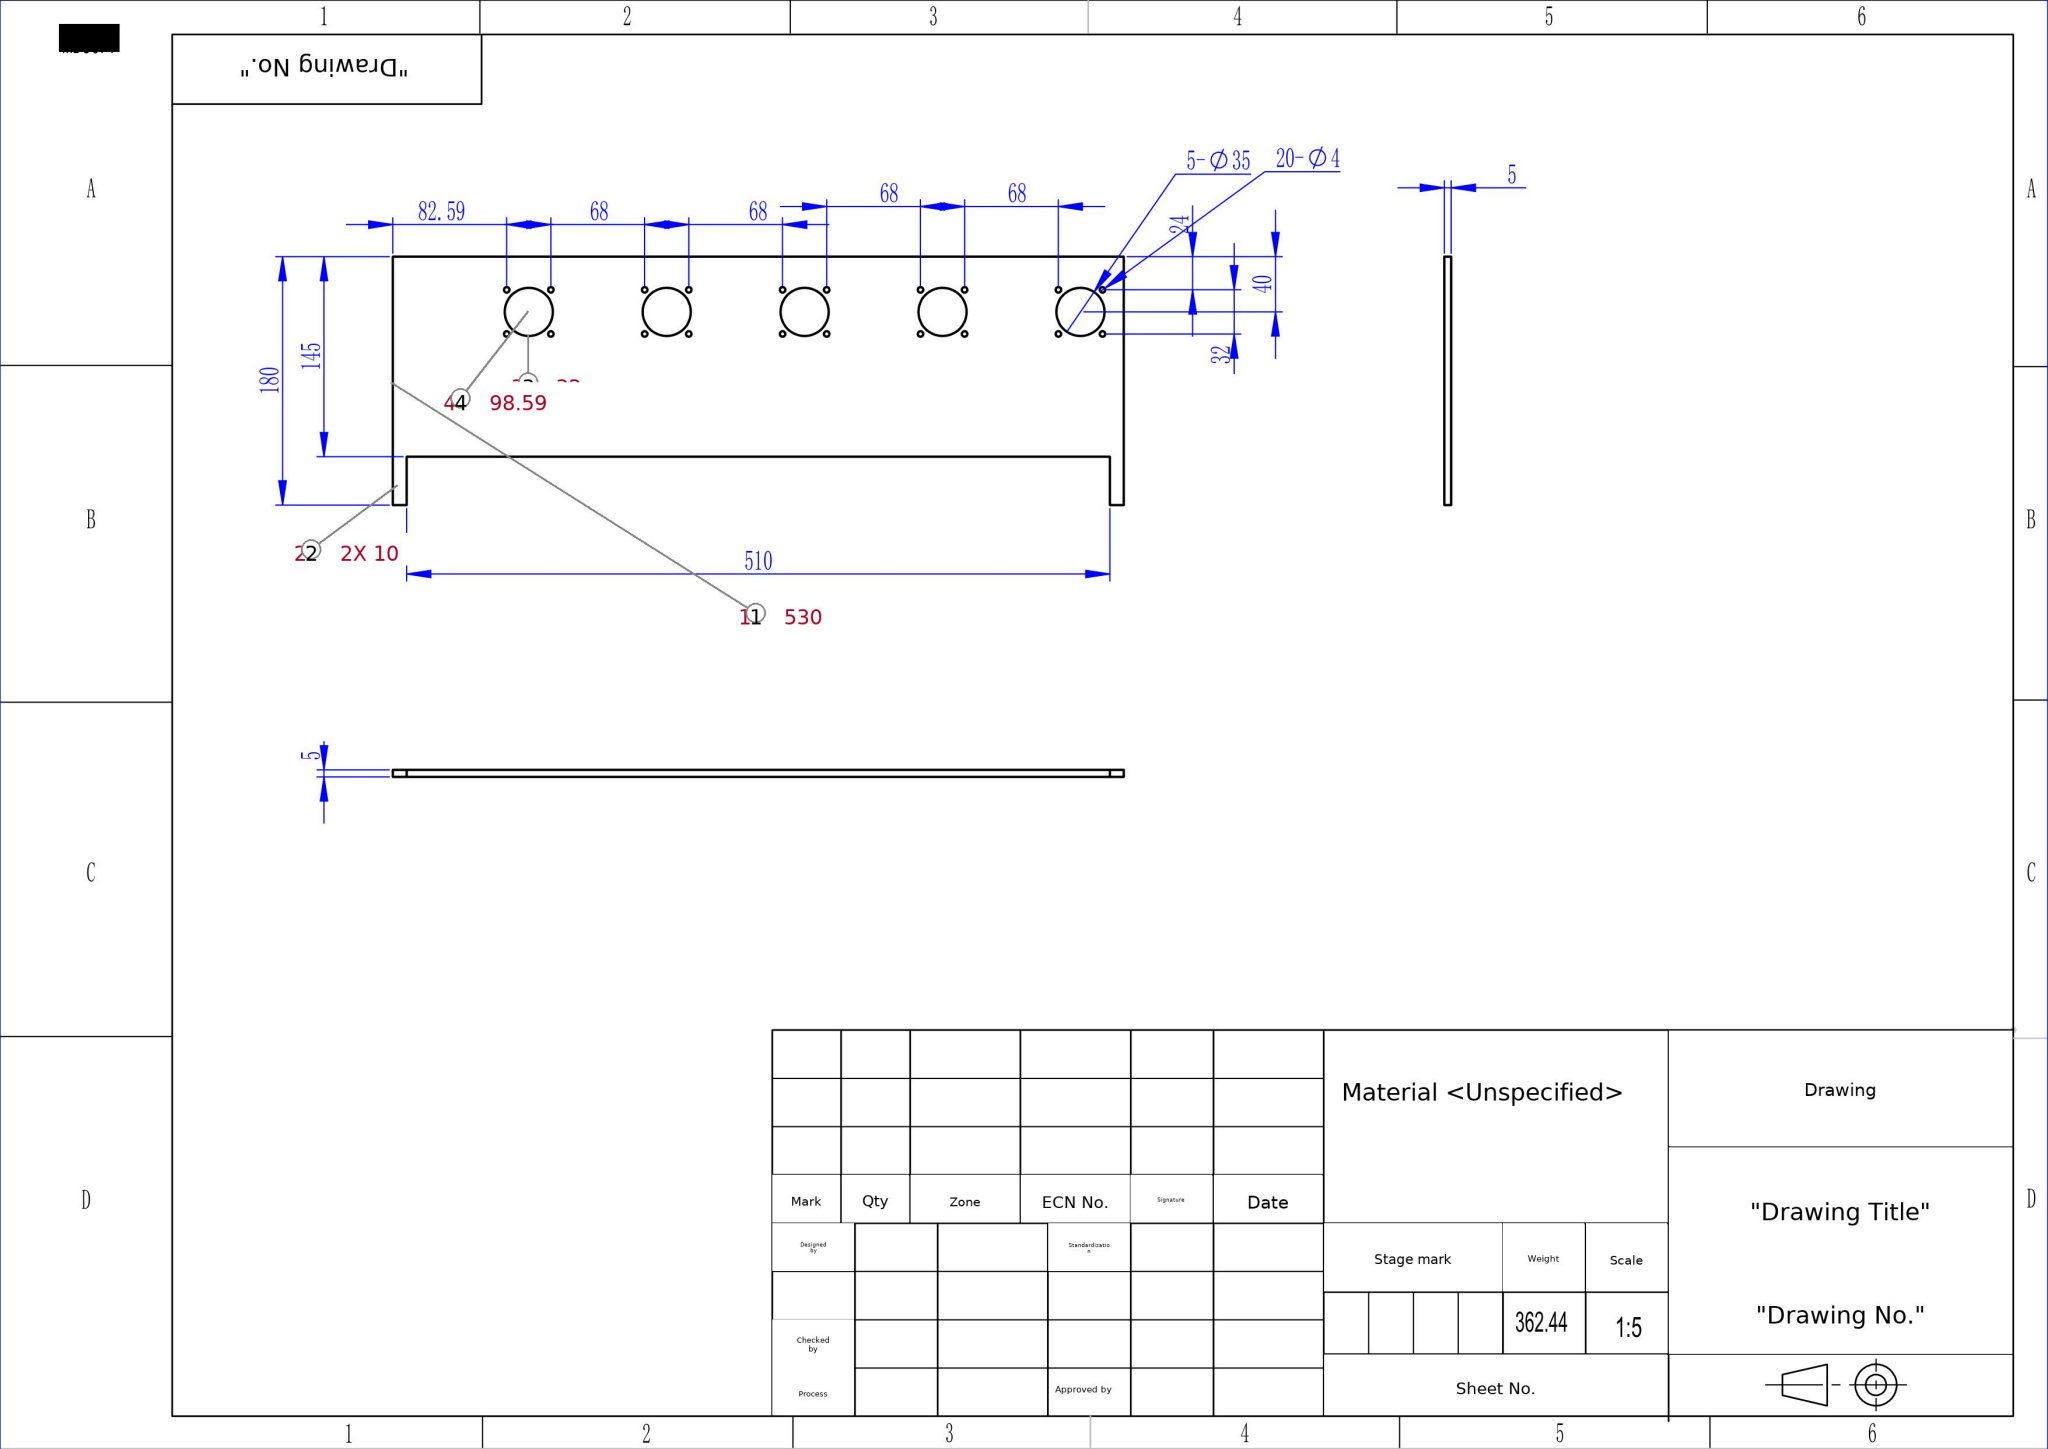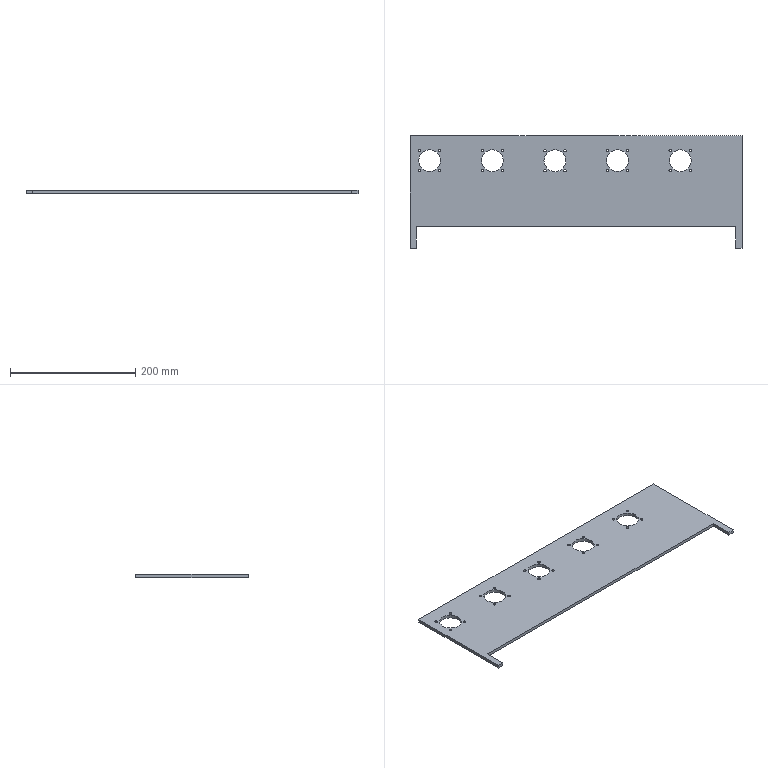Part | SolidWorks | mm | 1 solid | 60 faces | box 530 x 180 x 5 mm | volume 362441 mm3 | cylinder 50 | plane 10 | commonest cylinder face diameters 4 x40 35 x10
build123d program:
from build123d import *

# Parameters (mm, degrees)
SKETCH1_R           = 2
SKETCH1_R_2         = 17.5
BOSS_EXTRUDE1_DEPTH = 5


with BuildPart() as part:
    # Sketch1 → Boss-Extrude1 (new body)
    with BuildSketch(Plane.XY):
        Polygon((-265, 90), (265, 90), (265, -90), (255, -90), (255, -55), (-255, -55), (-255, -90), (-265, -90), align=None)
        with Locations((-249.585, 66)):
            Circle(SKETCH1_R, mode=Mode.SUBTRACT)
        with Locations((-217.585, 66)):
            Circle(SKETCH1_R, mode=Mode.SUBTRACT)
        with Locations((-217.585, 34)):
            Circle(SKETCH1_R, mode=Mode.SUBTRACT)
        with Locations((-249.585, 34)):
            Circle(SKETCH1_R, mode=Mode.SUBTRACT)
        with Locations((-233.585, 50)):
            Circle(SKETCH1_R_2, mode=Mode.SUBTRACT)
        with Locations((-149.585, 66)):
            Circle(SKETCH1_R, mode=Mode.SUBTRACT)
        with Locations((-117.585, 66)):
            Circle(SKETCH1_R, mode=Mode.SUBTRACT)
        with Locations((-117.585, 34)):
            Circle(SKETCH1_R, mode=Mode.SUBTRACT)
        with Locations((-149.585, 34)):
            Circle(SKETCH1_R, mode=Mode.SUBTRACT)
        with Locations((-133.585, 50)):
            Circle(SKETCH1_R_2, mode=Mode.SUBTRACT)
        with Locations((-49.585, 66)):
            Circle(SKETCH1_R, mode=Mode.SUBTRACT)
        with Locations((-17.585, 66)):
            Circle(SKETCH1_R, mode=Mode.SUBTRACT)
        with Locations((-17.585, 34)):
            Circle(SKETCH1_R, mode=Mode.SUBTRACT)
        with Locations((-49.585, 34)):
            Circle(SKETCH1_R, mode=Mode.SUBTRACT)
        with Locations((-33.585, 50)):
            Circle(SKETCH1_R_2, mode=Mode.SUBTRACT)
        with Locations((50.415, 66)):
            Circle(SKETCH1_R, mode=Mode.SUBTRACT)
        with Locations((82.415, 66)):
            Circle(SKETCH1_R, mode=Mode.SUBTRACT)
        with Locations((82.415, 34)):
            Circle(SKETCH1_R, mode=Mode.SUBTRACT)
        with Locations((50.415, 34)):
            Circle(SKETCH1_R, mode=Mode.SUBTRACT)
        with Locations((66.415, 50)):
            Circle(SKETCH1_R_2, mode=Mode.SUBTRACT)
        with Locations((150.415, 66)):
            Circle(SKETCH1_R, mode=Mode.SUBTRACT)
        with Locations((182.415, 66)):
            Circle(SKETCH1_R, mode=Mode.SUBTRACT)
        with Locations((182.415, 34)):
            Circle(SKETCH1_R, mode=Mode.SUBTRACT)
        with Locations((150.415, 34)):
            Circle(SKETCH1_R, mode=Mode.SUBTRACT)
        with Locations((166.415, 50)):
            Circle(SKETCH1_R_2, mode=Mode.SUBTRACT)
    extrude(amount=BOSS_EXTRUDE1_DEPTH)


solid = part.part